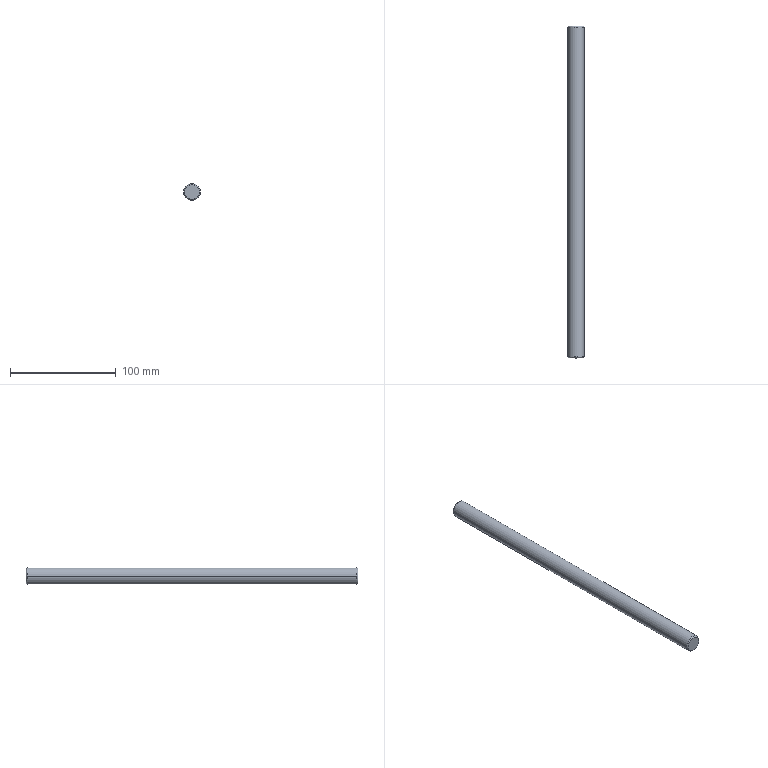Component | SolidWorks | NameDuplicate-1Slider-2 | 1 solid | 8 faces | box 16 x 314 x 16 mm | volume 63085 mm3 | cone 4 | cylinder 2 | plane 2 | commonest cylinder face diameters 16 x2
build123d program:
from build123d import *


with BuildPart() as part:
    # Sketch1 → Revolve1 (revolve)
    with BuildSketch(Plane(origin=(0, 0, 0), x_dir=(1, 0, 0), z_dir=(0, 1, 0))):
        Polygon((7, 157), (0, 157), (0, -157), (7, -157), (8, -156), (8, 156), align=None)
    revolve(axis=Axis((0, 0, -157), (0, 0, 1)))


solid = part.part

# Placed as in the assembly
solid = solid.moved(Location((-36, 54, -238.5), (90, 0, 0)))
STEP:
#1=CARTESIAN_POINT('',(-1.142,-4.055,-9.39));
#2=VERTEX_POINT('',#1);
#3=CARTESIAN_POINT('',(-1.693,-4.055,-9.39));
#4=VERTEX_POINT('',#3);
#5=CARTESIAN_POINT('',(-1.417,-4.055,-9.39));
#6=DIRECTION('',(-0.,-1.,0.));
#7=DIRECTION('',(1.,0.,0.));
#8=AXIS2_PLACEMENT_3D('',#5,#6,#7);
#9=CIRCLE('',#8,0.2756);
#10=EDGE_CURVE('',#2,#4,#9,.T.);
#11=ORIENTED_EDGE('',*,*,#10,.F.);
#12=CARTESIAN_POINT('',(-1.102,-4.016,-9.39));
#13=VERTEX_POINT('',#12);
#14=CARTESIAN_POINT('',(-1.142,-4.055,-9.39));
#15=DIRECTION('',(0.7071,0.7071,0.));
#16=VECTOR('',#15,39.37);
#17=LINE('',#14,#16);
#18=EDGE_CURVE('',#2,#13,#17,.T.);
#19=ORIENTED_EDGE('',*,*,#18,.T.);
#20=CARTESIAN_POINT('',(-1.732,-4.016,-9.39));
#21=VERTEX_POINT('',#20);
#22=CARTESIAN_POINT('',(-1.417,-4.016,-9.39));
#23=DIRECTION('',(-0.,-1.,0.));
#24=DIRECTION('',(1.,0.,0.));
#25=AXIS2_PLACEMENT_3D('',#22,#23,#24);
#26=CIRCLE('',#25,0.315);
#27=EDGE_CURVE('',#13,#21,#26,.T.);
#28=ORIENTED_EDGE('',*,*,#27,.T.);
#29=CARTESIAN_POINT('',(-1.693,-4.055,-9.39));
#30=DIRECTION('',(-0.7071,0.7071,-0.));
#31=VECTOR('',#30,39.37);
#32=LINE('',#29,#31);
#33=EDGE_CURVE('',#4,#21,#32,.T.);
#34=ORIENTED_EDGE('',*,*,#33,.F.);
#35=EDGE_LOOP('',(#11,#19,#28,#34));
#36=FACE_OUTER_BOUND('',#35,.T.);
#37=CARTESIAN_POINT('',(-1.417,-4.055,-9.39));
#38=DIRECTION('',(0.,1.,0.));
#39=DIRECTION('',(-1.,0.,0.));
#40=AXIS2_PLACEMENT_3D('',#37,#38,#39);
#41=CONICAL_SURFACE('',#40,0.2756,0.7854);
#42=ADVANCED_FACE('',(#36),#41,.T.);
#43=CARTESIAN_POINT('',(-1.102,8.268,-9.39));
#44=VERTEX_POINT('',#43);
#45=CARTESIAN_POINT('',(-1.732,8.268,-9.39));
#46=VERTEX_POINT('',#45);
#47=CARTESIAN_POINT('',(-1.417,8.268,-9.39));
#48=DIRECTION('',(-0.,-1.,0.));
#49=DIRECTION('',(1.,0.,0.));
#50=AXIS2_PLACEMENT_3D('',#47,#48,#49);
#51=CIRCLE('',#50,0.315);
#52=EDGE_CURVE('',#44,#46,#51,.T.);
#53=ORIENTED_EDGE('',*,*,#52,.T.);
#54=CARTESIAN_POINT('',(-1.732,8.307,-9.39));
#55=DIRECTION('',(-0.,-1.,0.));
#56=VECTOR('',#55,39.37);
#57=LINE('',#54,#56);
#58=EDGE_CURVE('',#46,#21,#57,.T.);
#59=ORIENTED_EDGE('',*,*,#58,.T.);
#60=ORIENTED_EDGE('',*,*,#27,.F.);
#61=CARTESIAN_POINT('',(-1.102,8.307,-9.39));
#62=DIRECTION('',(-0.,-1.,0.));
#63=VECTOR('',#62,39.37);
#64=LINE('',#61,#63);
#65=EDGE_CURVE('',#44,#13,#64,.T.);
#66=ORIENTED_EDGE('',*,*,#65,.F.);
#67=EDGE_LOOP('',(#53,#59,#60,#66));
#68=FACE_OUTER_BOUND('',#67,.T.);
#69=CARTESIAN_POINT('',(-1.417,8.307,-9.39));
#70=DIRECTION('',(-0.,-1.,0.));
#71=DIRECTION('',(1.,0.,0.));
#72=AXIS2_PLACEMENT_3D('',#69,#70,#71);
#73=CYLINDRICAL_SURFACE('',#72,0.315);
#74=ADVANCED_FACE('',(#68),#73,.T.);
#75=CARTESIAN_POINT('',(-1.142,8.307,-9.39));
#76=VERTEX_POINT('',#75);
#77=CARTESIAN_POINT('',(-1.693,8.307,-9.39));
#78=VERTEX_POINT('',#77);
#79=CARTESIAN_POINT('',(-1.417,8.307,-9.39));
#80=DIRECTION('',(-0.,-1.,0.));
#81=DIRECTION('',(1.,0.,0.));
#82=AXIS2_PLACEMENT_3D('',#79,#80,#81);
#83=CIRCLE('',#82,0.2756);
#84=EDGE_CURVE('',#76,#78,#83,.T.);
#85=ORIENTED_EDGE('',*,*,#84,.T.);
#86=CARTESIAN_POINT('',(-1.732,8.268,-9.39));
#87=DIRECTION('',(-0.7071,-0.7071,-0.));
#88=VECTOR('',#87,39.37);
#89=LINE('',#86,#88);
#90=EDGE_CURVE('',#78,#46,#89,.T.);
#91=ORIENTED_EDGE('',*,*,#90,.T.);
#92=ORIENTED_EDGE('',*,*,#52,.F.);
#93=CARTESIAN_POINT('',(-1.102,8.268,-9.39));
#94=DIRECTION('',(0.7071,-0.7071,0.));
#95=VECTOR('',#94,39.37);
#96=LINE('',#93,#95);
#97=EDGE_CURVE('',#76,#44,#96,.T.);
#98=ORIENTED_EDGE('',*,*,#97,.F.);
#99=EDGE_LOOP('',(#85,#91,#92,#98));
#100=FACE_OUTER_BOUND('',#99,.T.);
#101=CARTESIAN_POINT('',(-1.417,8.268,-9.39));
#102=DIRECTION('',(-0.,-1.,0.));
#103=DIRECTION('',(1.,0.,0.));
#104=AXIS2_PLACEMENT_3D('',#101,#102,#103);
#105=CONICAL_SURFACE('',#104,0.315,0.7854);
#106=ADVANCED_FACE('',(#100),#105,.T.);
#107=ORIENTED_EDGE('',*,*,#90,.F.);
#108=CARTESIAN_POINT('',(-1.417,8.307,-9.39));
#109=DIRECTION('',(-0.,-1.,0.));
#110=DIRECTION('',(1.,0.,0.));
#111=AXIS2_PLACEMENT_3D('',#108,#109,#110);
#112=CIRCLE('',#111,0.2756);
#113=EDGE_CURVE('',#78,#76,#112,.T.);
#114=ORIENTED_EDGE('',*,*,#113,.T.);
#115=ORIENTED_EDGE('',*,*,#97,.T.);
#116=CARTESIAN_POINT('',(-1.417,8.268,-9.39));
#117=DIRECTION('',(-0.,-1.,0.));
#118=DIRECTION('',(1.,0.,0.));
#119=AXIS2_PLACEMENT_3D('',#116,#117,#118);
#120=CIRCLE('',#119,0.315);
#121=EDGE_CURVE('',#46,#44,#120,.T.);
#122=ORIENTED_EDGE('',*,*,#121,.F.);
#123=EDGE_LOOP('',(#107,#114,#115,#122));
#124=FACE_OUTER_BOUND('',#123,.T.);
#125=CARTESIAN_POINT('',(-1.417,8.268,-9.39));
#126=DIRECTION('',(-0.,-1.,0.));
#127=DIRECTION('',(1.,0.,0.));
#128=AXIS2_PLACEMENT_3D('',#125,#126,#127);
#129=CONICAL_SURFACE('',#128,0.315,0.7854);
#130=ADVANCED_FACE('',(#124),#129,.T.);
#131=ORIENTED_EDGE('',*,*,#58,.F.);
#132=ORIENTED_EDGE('',*,*,#121,.T.);
#133=ORIENTED_EDGE('',*,*,#65,.T.);
#134=CARTESIAN_POINT('',(-1.417,-4.016,-9.39));
#135=DIRECTION('',(-0.,-1.,0.));
#136=DIRECTION('',(1.,0.,0.));
#137=AXIS2_PLACEMENT_3D('',#134,#135,#136);
#138=CIRCLE('',#137,0.315);
#139=EDGE_CURVE('',#21,#13,#138,.T.);
#140=ORIENTED_EDGE('',*,*,#139,.F.);
#141=EDGE_LOOP('',(#131,#132,#133,#140));
#142=FACE_OUTER_BOUND('',#141,.T.);
#143=CARTESIAN_POINT('',(-1.417,8.307,-9.39));
#144=DIRECTION('',(-0.,-1.,0.));
#145=DIRECTION('',(1.,0.,0.));
#146=AXIS2_PLACEMENT_3D('',#143,#144,#145);
#147=CYLINDRICAL_SURFACE('',#146,0.315);
#148=ADVANCED_FACE('',(#142),#147,.T.);
#149=ORIENTED_EDGE('',*,*,#18,.F.);
#150=CARTESIAN_POINT('',(-1.417,-4.055,-9.39));
#151=DIRECTION('',(-0.,-1.,0.));
#152=DIRECTION('',(1.,0.,0.));
#153=AXIS2_PLACEMENT_3D('',#150,#151,#152);
#154=CIRCLE('',#153,0.2756);
#155=EDGE_CURVE('',#4,#2,#154,.T.);
#156=ORIENTED_EDGE('',*,*,#155,.F.);
#157=ORIENTED_EDGE('',*,*,#33,.T.);
#158=ORIENTED_EDGE('',*,*,#139,.T.);
#159=EDGE_LOOP('',(#149,#156,#157,#158));
#160=FACE_OUTER_BOUND('',#159,.T.);
#161=CARTESIAN_POINT('',(-1.417,-4.055,-9.39));
#162=DIRECTION('',(0.,1.,0.));
#163=DIRECTION('',(-1.,0.,0.));
#164=AXIS2_PLACEMENT_3D('',#161,#162,#163);
#165=CONICAL_SURFACE('',#164,0.2756,0.7854);
#166=ADVANCED_FACE('',(#160),#165,.T.);
#167=ORIENTED_EDGE('',*,*,#155,.T.);
#168=ORIENTED_EDGE('',*,*,#10,.T.);
#169=EDGE_LOOP('',(#167,#168));
#170=FACE_OUTER_BOUND('',#169,.T.);
#171=CARTESIAN_POINT('',(-1.417,-4.055,-9.39));
#172=DIRECTION('',(-0.,-1.,0.));
#173=DIRECTION('',(1.,-0.,0.));
#174=AXIS2_PLACEMENT_3D('',#171,#172,#173);
#175=PLANE('',#174);
#176=ADVANCED_FACE('',(#170),#175,.T.);
#177=ORIENTED_EDGE('',*,*,#84,.F.);
#178=ORIENTED_EDGE('',*,*,#113,.F.);
#179=EDGE_LOOP('',(#177,#178));
#180=FACE_OUTER_BOUND('',#179,.T.);
#181=CARTESIAN_POINT('',(-1.142,8.307,-9.39));
#182=DIRECTION('',(0.,1.,0.));
#183=DIRECTION('',(-1.,0.,-0.));
#184=AXIS2_PLACEMENT_3D('',#181,#182,#183);
#185=PLANE('',#184);
#186=ADVANCED_FACE('',(#180),#185,.T.);
#187=CLOSED_SHELL('',(#42,#74,#106,#130,#148,#166,#176,#186));
#188=MANIFOLD_SOLID_BREP('',#187);
#189=CARTESIAN_POINT('',(0.,0.,0.));
#190=DIRECTION('',(0.,0.,1.));
#191=DIRECTION('',(1.,0.,0.));
#192=AXIS2_PLACEMENT_3D('',#189,#190,#191);
#193=(LENGTH_UNIT()NAMED_UNIT(*)SI_UNIT($,.METRE.));
#194=LENGTH_MEASURE_WITH_UNIT(LENGTH_MEASURE(0.0254),#193);
#195=DIMENSIONAL_EXPONENTS(1.,0.,0.,0.,0.,0.,0.);
#196=(CONVERSION_BASED_UNIT('',#194)LENGTH_UNIT()NAMED_UNIT(#195));
#197=UNCERTAINTY_MEASURE_WITH_UNIT(LENGTH_MEASURE(0.00001),#196,'','');
#198=(NAMED_UNIT(*)PLANE_ANGLE_UNIT()SI_UNIT($,.RADIAN.));
#199=(NAMED_UNIT(*)SI_UNIT($,.STERADIAN.)SOLID_ANGLE_UNIT());
#200=(GEOMETRIC_REPRESENTATION_CONTEXT(3)GLOBAL_UNCERTAINTY_ASSIGNED_CONTEXT((#197))GLOBAL_UNIT_ASSIGNED_CONTEXT((#196,#198,#199))REPRESENTATION_CONTEXT('',''));
#201=ADVANCED_BREP_SHAPE_REPRESENTATION('',(#188,#192),#200);
#202=COLOUR_RGB('',0.7922,0.8196,0.9333);
#203=FILL_AREA_STYLE_COLOUR('',#202);
#204=FILL_AREA_STYLE('',(#203));
#205=SURFACE_STYLE_FILL_AREA(#204);
#206=SURFACE_SIDE_STYLE('',(#205));
#207=SURFACE_STYLE_USAGE(.BOTH.,#206);
#208=PRESENTATION_STYLE_ASSIGNMENT((#207));
#209=STYLED_ITEM('',(#208),#188);
#210=PRESENTATION_LAYER_ASSIGNMENT('','',(#209));
#211=(LENGTH_UNIT()NAMED_UNIT(*)SI_UNIT($,.METRE.));
#212=LENGTH_MEASURE_WITH_UNIT(LENGTH_MEASURE(0.0254),#211);
#213=DIMENSIONAL_EXPONENTS(1.,0.,0.,0.,0.,0.,0.);
#214=(CONVERSION_BASED_UNIT('',#212)LENGTH_UNIT()NAMED_UNIT(#213));
#215=UNCERTAINTY_MEASURE_WITH_UNIT(LENGTH_MEASURE(0.00001),#214,'','');
#216=(NAMED_UNIT(*)PLANE_ANGLE_UNIT()SI_UNIT($,.RADIAN.));
#217=(NAMED_UNIT(*)SI_UNIT($,.STERADIAN.)SOLID_ANGLE_UNIT());
#218=(GEOMETRIC_REPRESENTATION_CONTEXT(3)GLOBAL_UNCERTAINTY_ASSIGNED_CONTEXT((#215))GLOBAL_UNIT_ASSIGNED_CONTEXT((#214,#216,#217))REPRESENTATION_CONTEXT('',''));
#219=MECHANICAL_DESIGN_GEOMETRIC_PRESENTATION_REPRESENTATION('',(#209),#218);